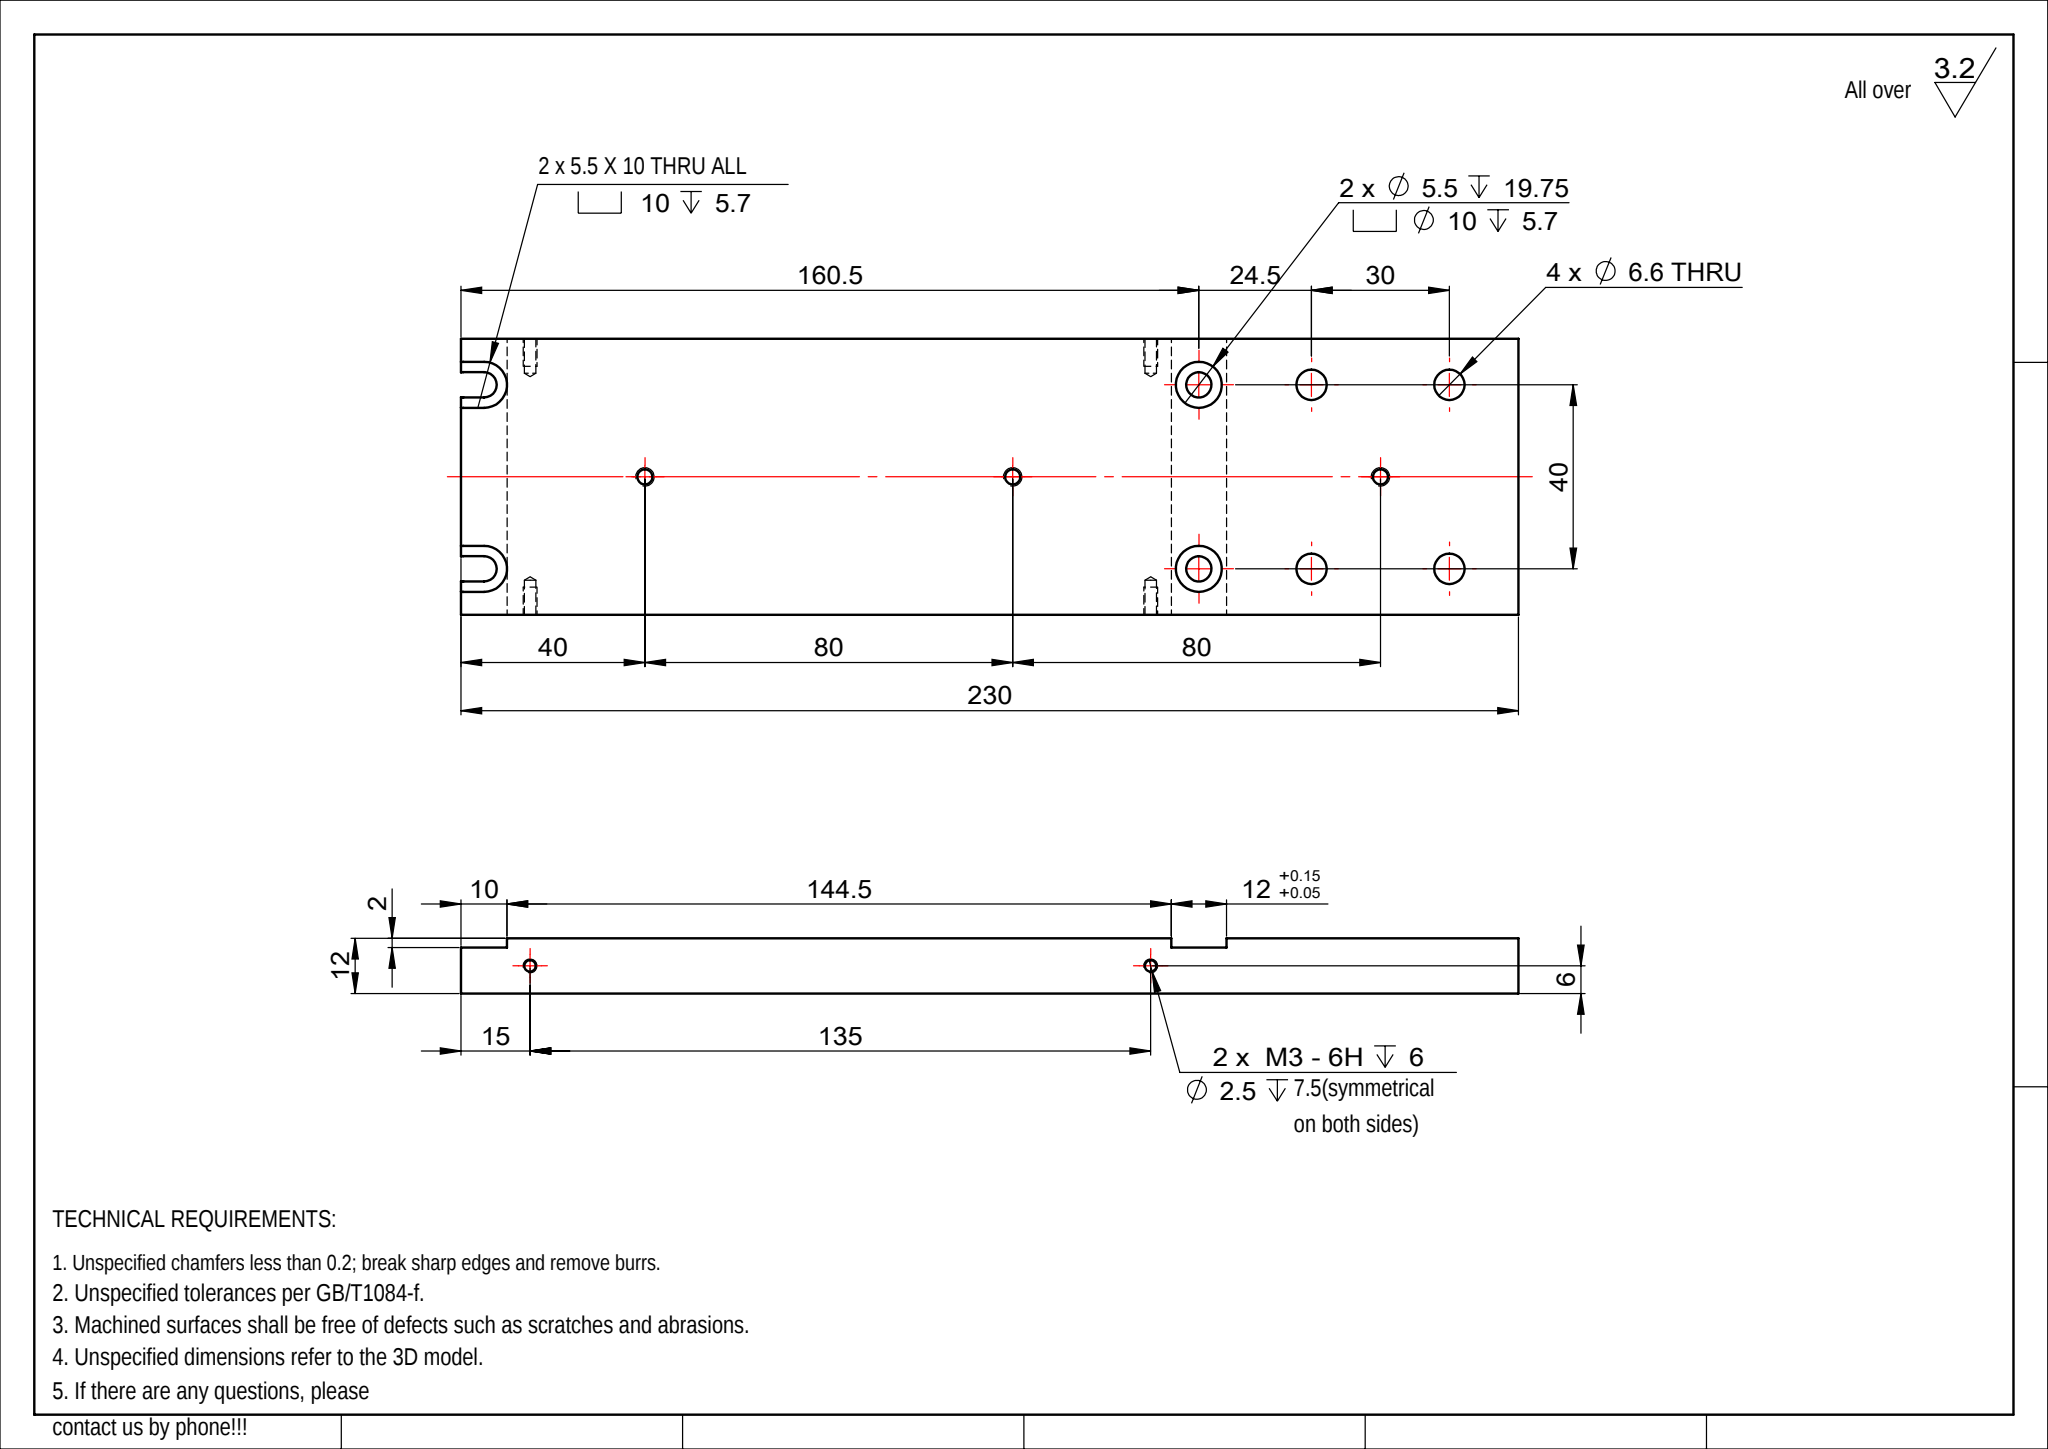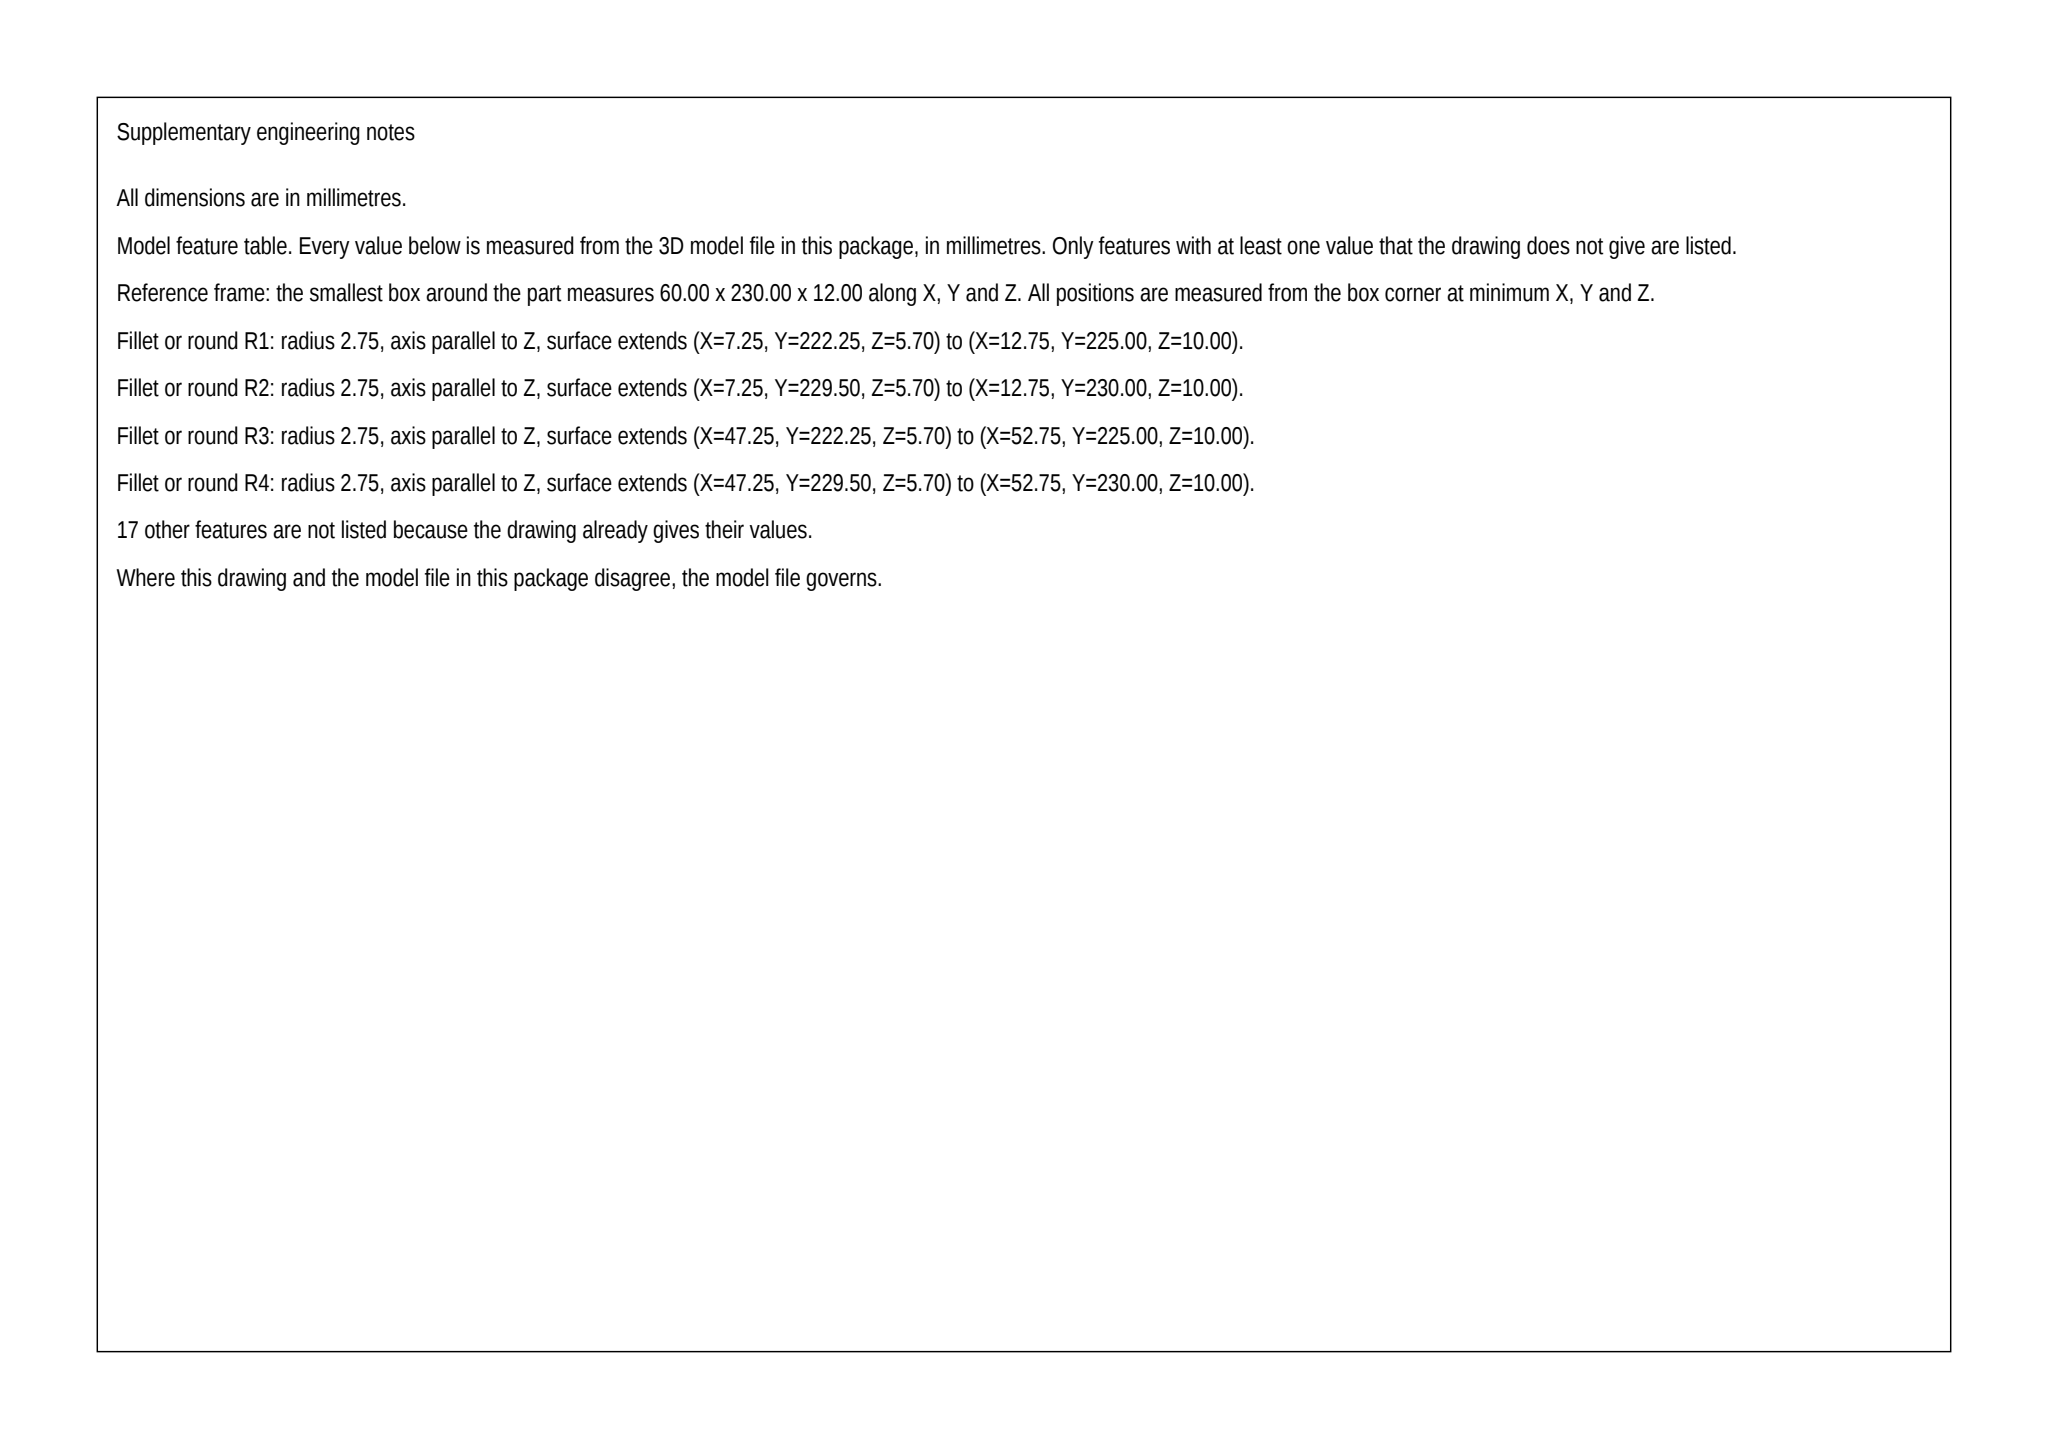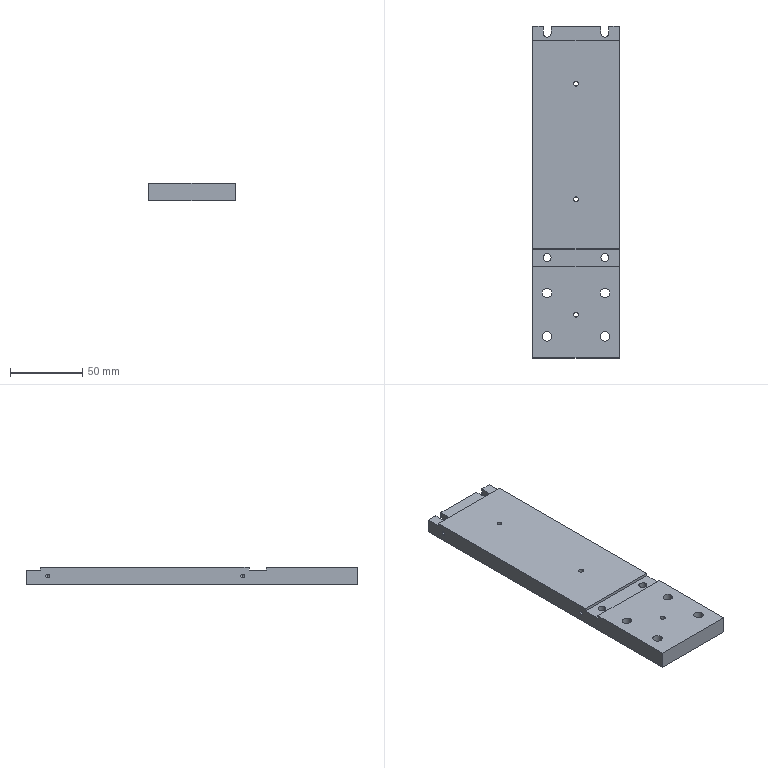Part | SolidWorks | mm | 1 solid | 76 faces | box 60 x 230 x 12 mm | volume 158402 mm3 | cylinder 42 | plane 26 | cone 8 | commonest cylinder face diameters 10 x10 5.5 x10 6.6 x8 2.5 x8 3.3 x6